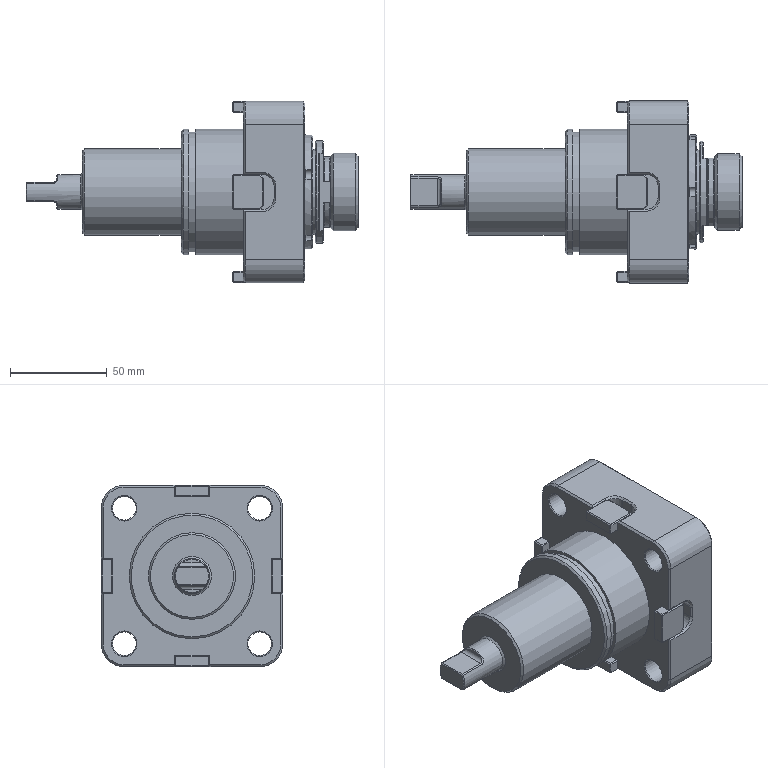Component | NX | 12_01_BODY | 1 solid | 290 faces | volume 469506 mm3 | plane 190 | cone 54 | cylinder 39 | spline 4 | torus 3 | commonest cylinder face diameters 12 x8 24 x5 5 x5 12.2 x4 18.4 x4 36.6 x2 64.9 x2 4 x2